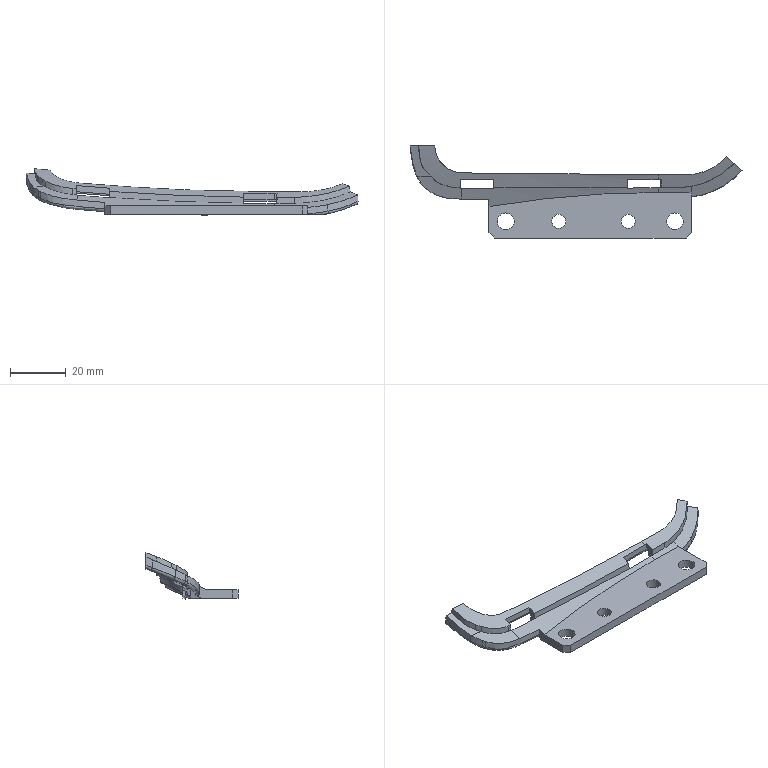CAM job | NX | mm | 3-axis | 1 set-up | 2 operations | part box 119.16 x 33.02 x 16.68
set-up 1
1. Cavity Milling | Mill Mill5 DB-20R5 | CAVITY_MILL | path 88269.216 mm | 29.39 min
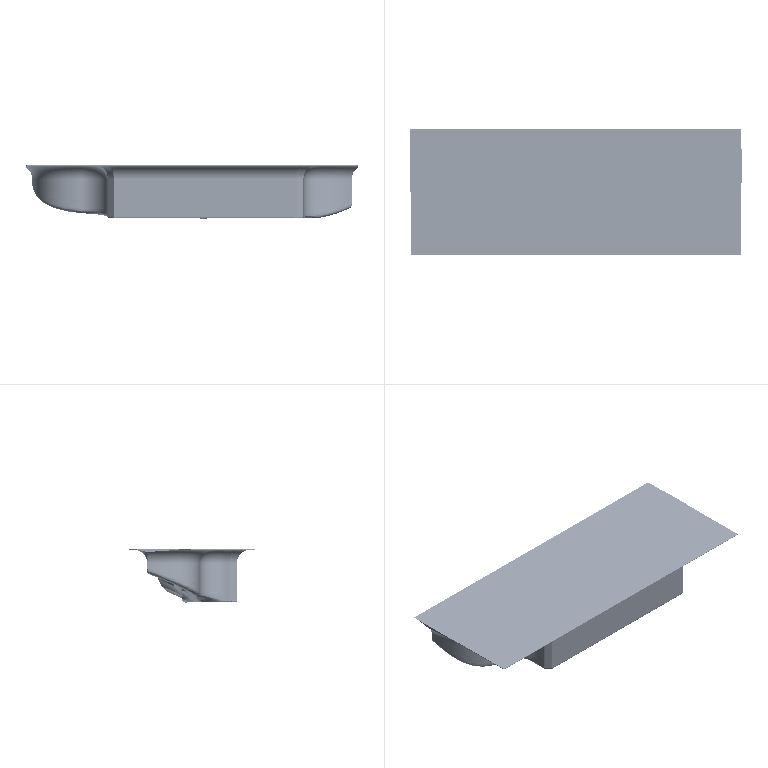2. Cavity Milling | Mill Mill5 DA-8 | CAVITY_MILL_COPY | path 13731.397 mm | 3.236 min